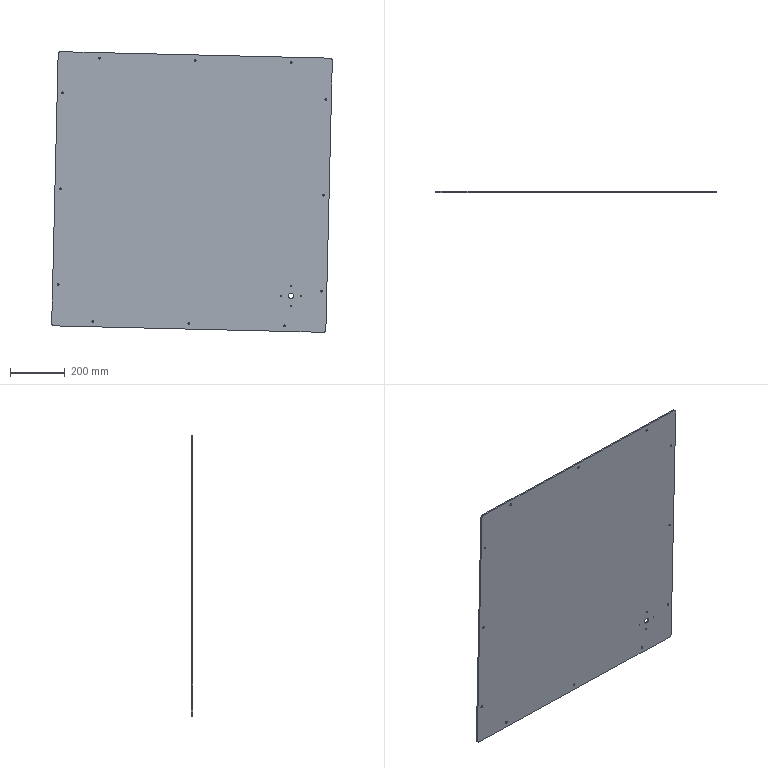Component | SolidWorks | 2012MB0201-1_UpperRackCoverModule-1_A3009-1 | 1 solid | 68 faces | volume 4994211 mm3 | cylinder 38 | cone 24 | plane 6 | commonest cylinder face diameters 6.6 x24 4.2 x8 20 x6 | material PC